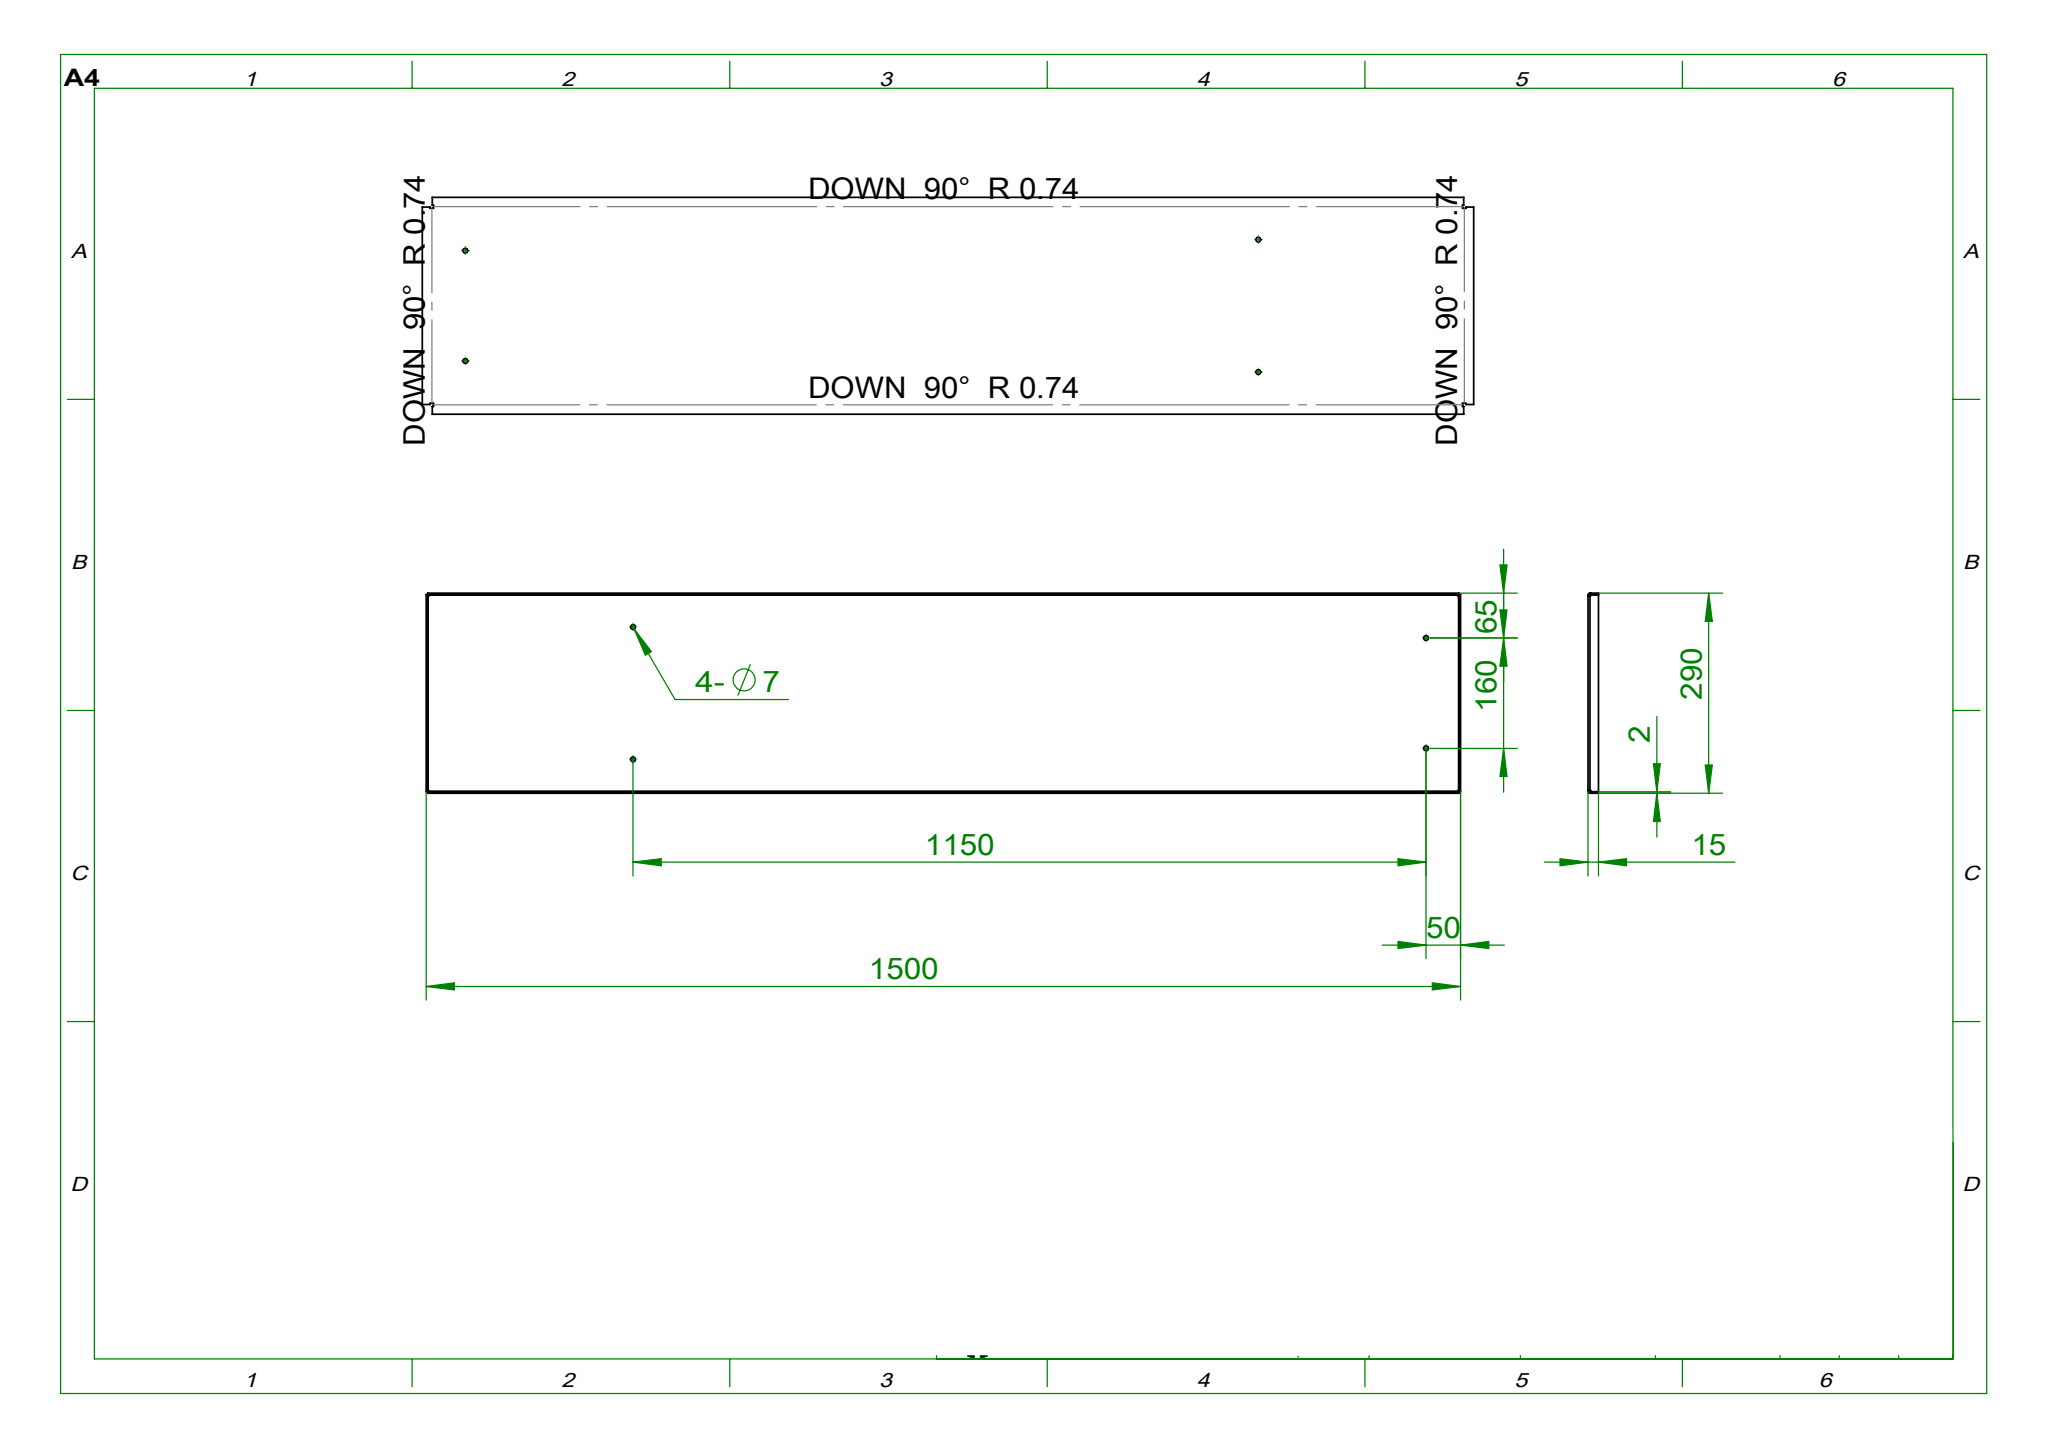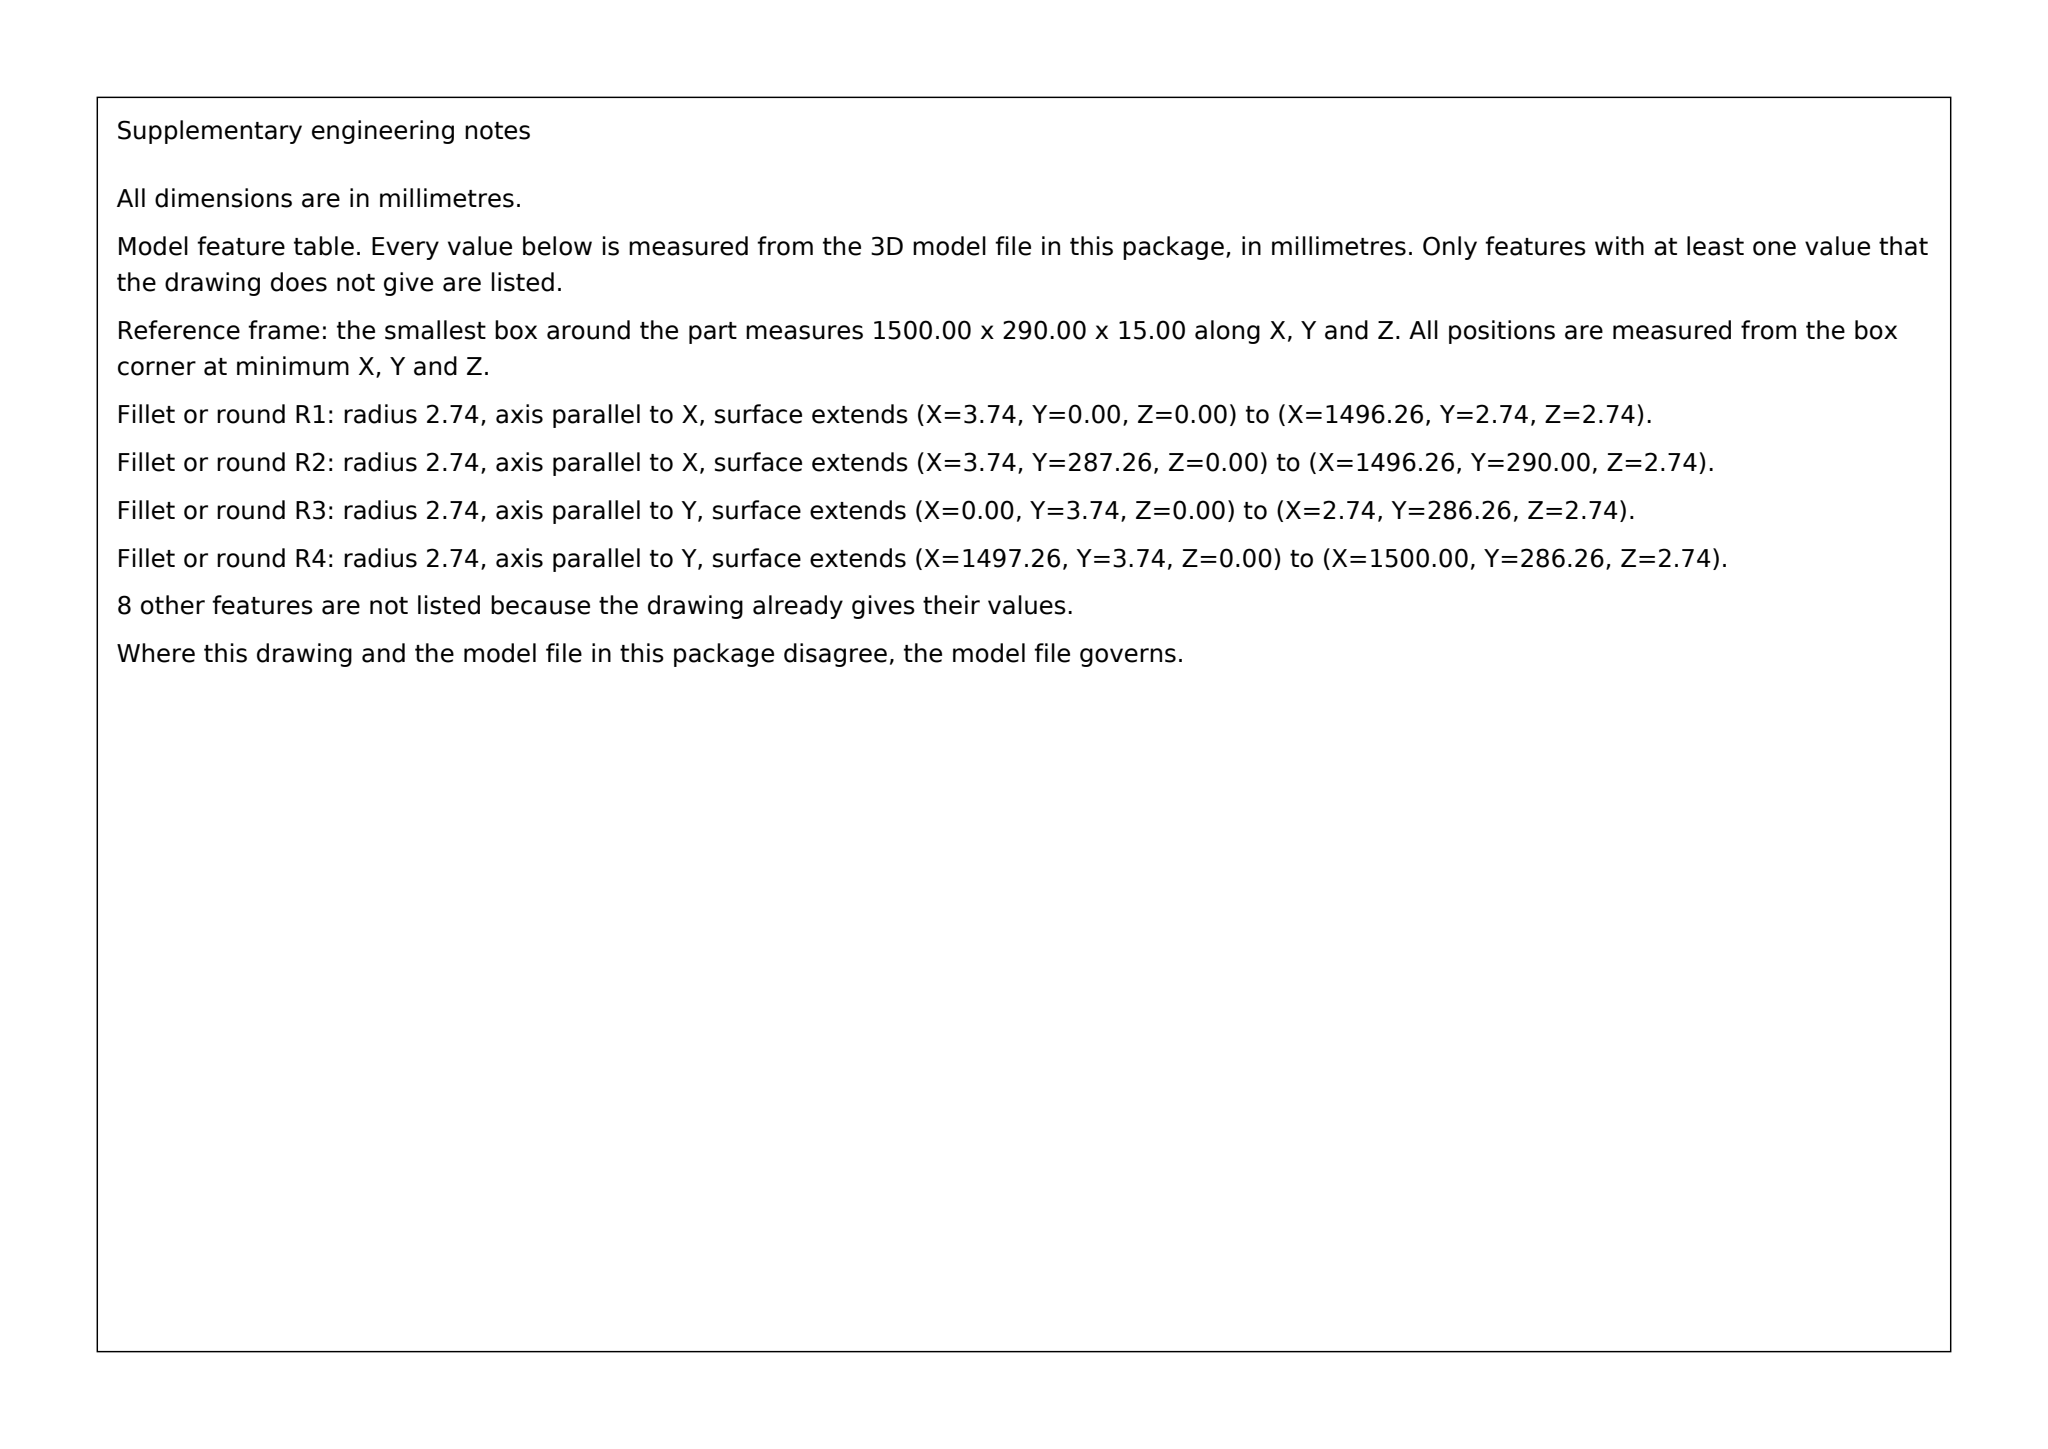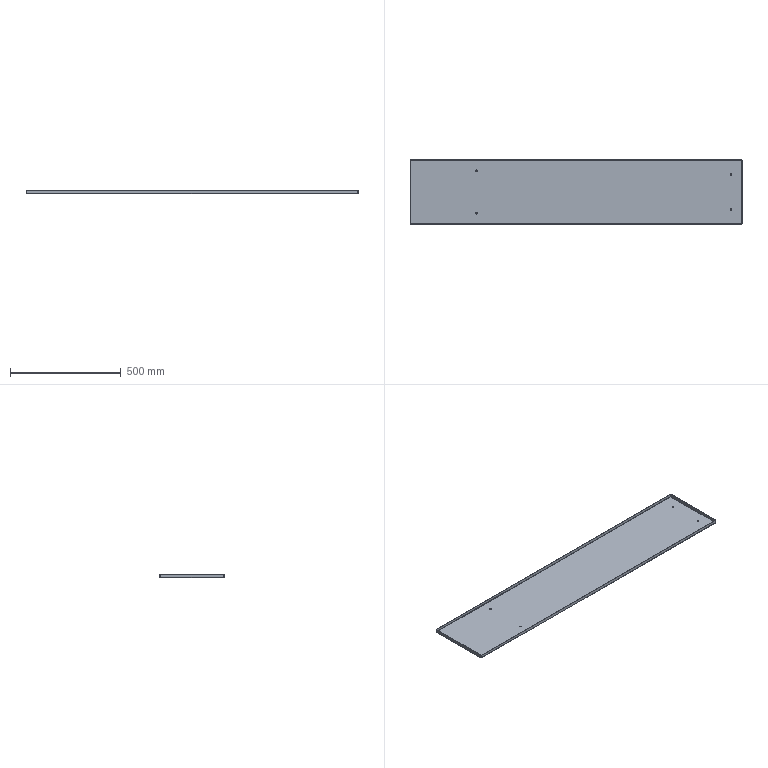Part | SolidWorks | mm | 1 solid | 70 faces | box 1500 x 290 x 15 mm | volume 956891 mm3 | plane 54 | cylinder 16 | commonest cylinder face diameters 7 x8 5.473 x4 1.473 x4
Drawing notes:
LH 2X Ø7 HOLES AT Y=49.02 & 240.98 FROM LOWER EDGE | from the solid: cylinders dia 7, axis z, pos [300, 49.02] and [300, 240.98]
HOLE PATTERN NOT SYM: LH PAIR 49.02 EDGE DIST, 191.96 APART | from the solid: LH holes y=49.02/240.98 (290-240.98=49.02, spacing 191.96) vs RH y=65/225